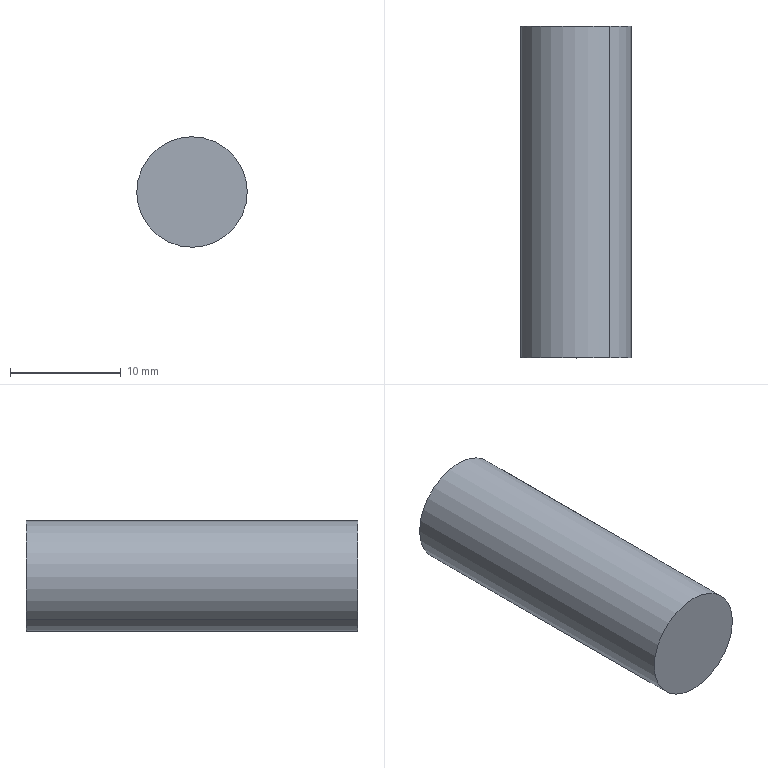Component | SolidWorks | 05-1 | 1 solid | 7 faces | box 10 x 30 x 10 mm | volume 2219 mm3 | cylinder 4 | plane 3 | commonest cylinder face diameters 5 x2 10 x2
build123d program:
from build123d import *

# Parameters (mm, degrees)
SKETCH1_2_R             = 5
BOSS_EXTRUDE1_DEPTH     = 30
SKETCH1_R               = 2.5
M5_TAP_CDU_RODEND_DEPTH = 7


with BuildPart() as part:
    # Sketch1_2 → Boss-Extrude1 (new body)
    with BuildSketch(Plane.XY):
        Circle(SKETCH1_2_R)
    extrude(amount=BOSS_EXTRUDE1_DEPTH)

    # Sketch1 → M5_Tap_CDU_RodEnd (cut)
    with BuildSketch(Plane.XY.offset(30)):
        Circle(SKETCH1_R)
    extrude(amount=-M5_TAP_CDU_RODEND_DEPTH, mode=Mode.SUBTRACT)


solid = part.part

# Placed as in the assembly
solid = solid.moved(Location((-42, 120.3, 116), (-90, 0, 0)))
STEP:
#1=COLOUR_RGB('',0.7922,0.8196,0.9333);
#2=FILL_AREA_STYLE_COLOUR('',#1);
#3=FILL_AREA_STYLE('',(#2));
#4=SURFACE_STYLE_FILL_AREA(#3);
#5=SURFACE_SIDE_STYLE('',(#4));
#6=SURFACE_STYLE_USAGE(.BOTH.,#5);
#7=PRESENTATION_STYLE_ASSIGNMENT((#6));
#8=CARTESIAN_POINT('',(-1.593,5.642,4.645));
#9=VERTEX_POINT('',#8);
#10=CARTESIAN_POINT('',(-1.714,5.642,4.489));
#11=VERTEX_POINT('',#10);
#12=CARTESIAN_POINT('',(-1.654,5.642,4.567));
#13=DIRECTION('',(0.,1.,-0.));
#14=DIRECTION('',(-0.6141,0.,-0.7892));
#15=AXIS2_PLACEMENT_3D('',#12,#13,#14);
#16=CIRCLE('',#15,0.09843);
#17=EDGE_CURVE('',#9,#11,#16,.T.);
#18=ORIENTED_EDGE('',*,*,#17,.F.);
#19=CARTESIAN_POINT('',(-1.593,5.917,4.645));
#20=VERTEX_POINT('',#19);
#21=CARTESIAN_POINT('',(-1.593,5.642,4.645));
#22=DIRECTION('',(0.,1.,-0.));
#23=VECTOR('',#22,39.37);
#24=LINE('',#21,#23);
#25=EDGE_CURVE('',#9,#20,#24,.T.);
#26=ORIENTED_EDGE('',*,*,#25,.T.);
#27=CARTESIAN_POINT('',(-1.714,5.917,4.489));
#28=VERTEX_POINT('',#27);
#29=CARTESIAN_POINT('',(-1.654,5.917,4.567));
#30=DIRECTION('',(0.,1.,-0.));
#31=DIRECTION('',(-0.6141,0.,-0.7892));
#32=AXIS2_PLACEMENT_3D('',#29,#30,#31);
#33=CIRCLE('',#32,0.09843);
#34=EDGE_CURVE('',#20,#28,#33,.T.);
#35=ORIENTED_EDGE('',*,*,#34,.T.);
#36=CARTESIAN_POINT('',(-1.714,5.642,4.489));
#37=DIRECTION('',(0.,1.,-0.));
#38=VECTOR('',#37,39.37);
#39=LINE('',#36,#38);
#40=EDGE_CURVE('',#11,#28,#39,.T.);
#41=ORIENTED_EDGE('',*,*,#40,.F.);
#42=EDGE_LOOP('',(#18,#26,#35,#41));
#43=FACE_OUTER_BOUND('',#42,.T.);
#44=CARTESIAN_POINT('',(-1.654,5.642,4.567));
#45=DIRECTION('',(0.,1.,-0.));
#46=DIRECTION('',(-0.6141,0.,-0.7892));
#47=AXIS2_PLACEMENT_3D('',#44,#45,#46);
#48=CYLINDRICAL_SURFACE('',#47,0.09843);
#49=ADVANCED_FACE('',(#43),#48,.F.);
#50=CARTESIAN_POINT('',(-1.774,5.917,4.412));
#51=VERTEX_POINT('',#50);
#52=CARTESIAN_POINT('',(-1.533,5.917,4.722));
#53=VERTEX_POINT('',#52);
#54=CARTESIAN_POINT('',(-1.654,5.917,4.567));
#55=DIRECTION('',(0.,1.,-0.));
#56=DIRECTION('',(-0.6141,0.,-0.7892));
#57=AXIS2_PLACEMENT_3D('',#54,#55,#56);
#58=CIRCLE('',#57,0.1969);
#59=EDGE_CURVE('',#51,#53,#58,.T.);
#60=ORIENTED_EDGE('',*,*,#59,.F.);
#61=CARTESIAN_POINT('',(-1.774,4.736,4.412));
#62=VERTEX_POINT('',#61);
#63=CARTESIAN_POINT('',(-1.774,5.917,4.412));
#64=DIRECTION('',(-0.,-1.,0.));
#65=VECTOR('',#64,39.37);
#66=LINE('',#63,#65);
#67=EDGE_CURVE('',#51,#62,#66,.T.);
#68=ORIENTED_EDGE('',*,*,#67,.T.);
#69=CARTESIAN_POINT('',(-1.533,4.736,4.722));
#70=VERTEX_POINT('',#69);
#71=CARTESIAN_POINT('',(-1.654,4.736,4.567));
#72=DIRECTION('',(0.,1.,-0.));
#73=DIRECTION('',(-0.6141,0.,-0.7892));
#74=AXIS2_PLACEMENT_3D('',#71,#72,#73);
#75=CIRCLE('',#74,0.1969);
#76=EDGE_CURVE('',#62,#70,#75,.T.);
#77=ORIENTED_EDGE('',*,*,#76,.T.);
#78=CARTESIAN_POINT('',(-1.533,5.917,4.722));
#79=DIRECTION('',(-0.,-1.,0.));
#80=VECTOR('',#79,39.37);
#81=LINE('',#78,#80);
#82=EDGE_CURVE('',#53,#70,#81,.T.);
#83=ORIENTED_EDGE('',*,*,#82,.F.);
#84=EDGE_LOOP('',(#60,#68,#77,#83));
#85=FACE_OUTER_BOUND('',#84,.T.);
#86=CARTESIAN_POINT('',(-1.654,5.917,4.567));
#87=DIRECTION('',(-0.,-1.,0.));
#88=DIRECTION('',(0.6141,0.,0.7892));
#89=AXIS2_PLACEMENT_3D('',#86,#87,#88);
#90=CYLINDRICAL_SURFACE('',#89,0.1969);
#91=ADVANCED_FACE('',(#85),#90,.T.);
#92=ORIENTED_EDGE('',*,*,#67,.F.);
#93=CARTESIAN_POINT('',(-1.654,5.917,4.567));
#94=DIRECTION('',(0.,1.,-0.));
#95=DIRECTION('',(-0.6141,0.,-0.7892));
#96=AXIS2_PLACEMENT_3D('',#93,#94,#95);
#97=CIRCLE('',#96,0.1969);
#98=EDGE_CURVE('',#53,#51,#97,.T.);
#99=ORIENTED_EDGE('',*,*,#98,.F.);
#100=ORIENTED_EDGE('',*,*,#82,.T.);
#101=CARTESIAN_POINT('',(-1.654,4.736,4.567));
#102=DIRECTION('',(0.,1.,-0.));
#103=DIRECTION('',(-0.6141,0.,-0.7892));
#104=AXIS2_PLACEMENT_3D('',#101,#102,#103);
#105=CIRCLE('',#104,0.1969);
#106=EDGE_CURVE('',#70,#62,#105,.T.);
#107=ORIENTED_EDGE('',*,*,#106,.T.);
#108=EDGE_LOOP('',(#92,#99,#100,#107));
#109=FACE_OUTER_BOUND('',#108,.T.);
#110=CARTESIAN_POINT('',(-1.654,5.917,4.567));
#111=DIRECTION('',(-0.,-1.,0.));
#112=DIRECTION('',(0.6141,0.,0.7892));
#113=AXIS2_PLACEMENT_3D('',#110,#111,#112);
#114=CYLINDRICAL_SURFACE('',#113,0.1969);
#115=ADVANCED_FACE('',(#109),#114,.T.);
#116=CARTESIAN_POINT('',(-1.654,5.917,4.567));
#117=DIRECTION('',(0.,1.,-0.));
#118=DIRECTION('',(-0.6141,0.,-0.7892));
#119=AXIS2_PLACEMENT_3D('',#116,#117,#118);
#120=CIRCLE('',#119,0.09843);
#121=EDGE_CURVE('',#28,#20,#120,.T.);
#122=ORIENTED_EDGE('',*,*,#121,.F.);
#123=ORIENTED_EDGE('',*,*,#34,.F.);
#124=EDGE_LOOP('',(#122,#123));
#125=FACE_BOUND('',#124,.T.);
#126=ORIENTED_EDGE('',*,*,#98,.T.);
#127=ORIENTED_EDGE('',*,*,#59,.T.);
#128=EDGE_LOOP('',(#126,#127));
#129=FACE_OUTER_BOUND('',#128,.T.);
#130=CARTESIAN_POINT('',(-1.654,5.917,4.567));
#131=DIRECTION('',(0.,1.,-0.));
#132=DIRECTION('',(-0.6141,-0.,-0.7892));
#133=AXIS2_PLACEMENT_3D('',#130,#131,#132);
#134=PLANE('',#133);
#135=ADVANCED_FACE('',(#125,#129),#134,.T.);
#136=ORIENTED_EDGE('',*,*,#106,.F.);
#137=ORIENTED_EDGE('',*,*,#76,.F.);
#138=EDGE_LOOP('',(#136,#137));
#139=FACE_OUTER_BOUND('',#138,.T.);
#140=CARTESIAN_POINT('',(-1.654,4.736,4.567));
#141=DIRECTION('',(0.,1.,-0.));
#142=DIRECTION('',(-0.6141,-0.,-0.7892));
#143=AXIS2_PLACEMENT_3D('',#140,#141,#142);
#144=PLANE('',#143);
#145=ADVANCED_FACE('',(#139),#144,.F.);
#146=ORIENTED_EDGE('',*,*,#25,.F.);
#147=CARTESIAN_POINT('',(-1.654,5.642,4.567));
#148=DIRECTION('',(0.,1.,-0.));
#149=DIRECTION('',(-0.6141,0.,-0.7892));
#150=AXIS2_PLACEMENT_3D('',#147,#148,#149);
#151=CIRCLE('',#150,0.09843);
#152=EDGE_CURVE('',#11,#9,#151,.T.);
#153=ORIENTED_EDGE('',*,*,#152,.F.);
#154=ORIENTED_EDGE('',*,*,#40,.T.);
#155=ORIENTED_EDGE('',*,*,#121,.T.);
#156=EDGE_LOOP('',(#146,#153,#154,#155));
#157=FACE_OUTER_BOUND('',#156,.T.);
#158=CARTESIAN_POINT('',(-1.654,5.642,4.567));
#159=DIRECTION('',(0.,1.,-0.));
#160=DIRECTION('',(-0.6141,0.,-0.7892));
#161=AXIS2_PLACEMENT_3D('',#158,#159,#160);
#162=CYLINDRICAL_SURFACE('',#161,0.09843);
#163=ADVANCED_FACE('',(#157),#162,.F.);
#164=ORIENTED_EDGE('',*,*,#152,.T.);
#165=ORIENTED_EDGE('',*,*,#17,.T.);
#166=EDGE_LOOP('',(#164,#165));
#167=FACE_OUTER_BOUND('',#166,.T.);
#168=CARTESIAN_POINT('',(-1.654,5.642,4.567));
#169=DIRECTION('',(0.,1.,-0.));
#170=DIRECTION('',(-0.6141,-0.,-0.7892));
#171=AXIS2_PLACEMENT_3D('',#168,#169,#170);
#172=PLANE('',#171);
#173=ADVANCED_FACE('',(#167),#172,.T.);
#174=CLOSED_SHELL('',(#49,#91,#115,#135,#145,#163,#173));
#175=MANIFOLD_SOLID_BREP('',#174);
#176=STYLED_ITEM('',(#7),#175);
#177=(LENGTH_UNIT()NAMED_UNIT(*)SI_UNIT($,.METRE.));
#178=LENGTH_MEASURE_WITH_UNIT(LENGTH_MEASURE(0.0254),#177);
#179=DIMENSIONAL_EXPONENTS(1.,0.,0.,0.,0.,0.,0.);
#180=(CONVERSION_BASED_UNIT('',#178)LENGTH_UNIT()NAMED_UNIT(#179));
#181=UNCERTAINTY_MEASURE_WITH_UNIT(LENGTH_MEASURE(0.00001),#180,'','');
#182=(NAMED_UNIT(*)PLANE_ANGLE_UNIT()SI_UNIT($,.RADIAN.));
#183=(NAMED_UNIT(*)SI_UNIT($,.STERADIAN.)SOLID_ANGLE_UNIT());
#184=(GEOMETRIC_REPRESENTATION_CONTEXT(3)GLOBAL_UNCERTAINTY_ASSIGNED_CONTEXT((#181))GLOBAL_UNIT_ASSIGNED_CONTEXT((#180,#182,#183))REPRESENTATION_CONTEXT('',''));
#185=MECHANICAL_DESIGN_GEOMETRIC_PRESENTATION_REPRESENTATION('',(#176),#184);
#186=CARTESIAN_POINT('',(0.,0.,0.));
#187=DIRECTION('',(0.,0.,1.));
#188=DIRECTION('',(1.,0.,0.));
#189=AXIS2_PLACEMENT_3D('',#186,#187,#188);
#190=(LENGTH_UNIT()NAMED_UNIT(*)SI_UNIT($,.METRE.));
#191=LENGTH_MEASURE_WITH_UNIT(LENGTH_MEASURE(0.0254),#190);
#192=DIMENSIONAL_EXPONENTS(1.,0.,0.,0.,0.,0.,0.);
#193=(CONVERSION_BASED_UNIT('',#191)LENGTH_UNIT()NAMED_UNIT(#192));
#194=UNCERTAINTY_MEASURE_WITH_UNIT(LENGTH_MEASURE(0.00001),#193,'','');
#195=(NAMED_UNIT(*)PLANE_ANGLE_UNIT()SI_UNIT($,.RADIAN.));
#196=(NAMED_UNIT(*)SI_UNIT($,.STERADIAN.)SOLID_ANGLE_UNIT());
#197=(GEOMETRIC_REPRESENTATION_CONTEXT(3)GLOBAL_UNCERTAINTY_ASSIGNED_CONTEXT((#194))GLOBAL_UNIT_ASSIGNED_CONTEXT((#193,#195,#196))REPRESENTATION_CONTEXT('',''));
#198=ADVANCED_BREP_SHAPE_REPRESENTATION('',(#175,#189),#197);
#199=PRESENTATION_LAYER_ASSIGNMENT('','',(#176));